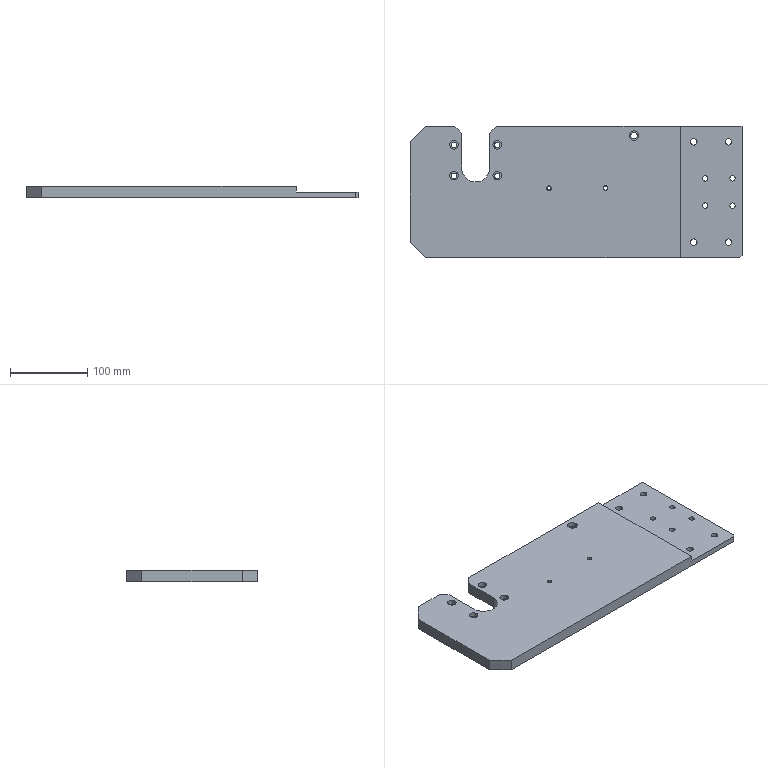Component | SolidWorks | BottomPlate(1)-1 | 1 solid | 66 faces | volume 942093 mm3 | cylinder 41 | plane 21 | cone 4 | commonest cylinder face diameters 7 x16 8.5 x10 11 x8 5 x4 12.5 x2 36 x1